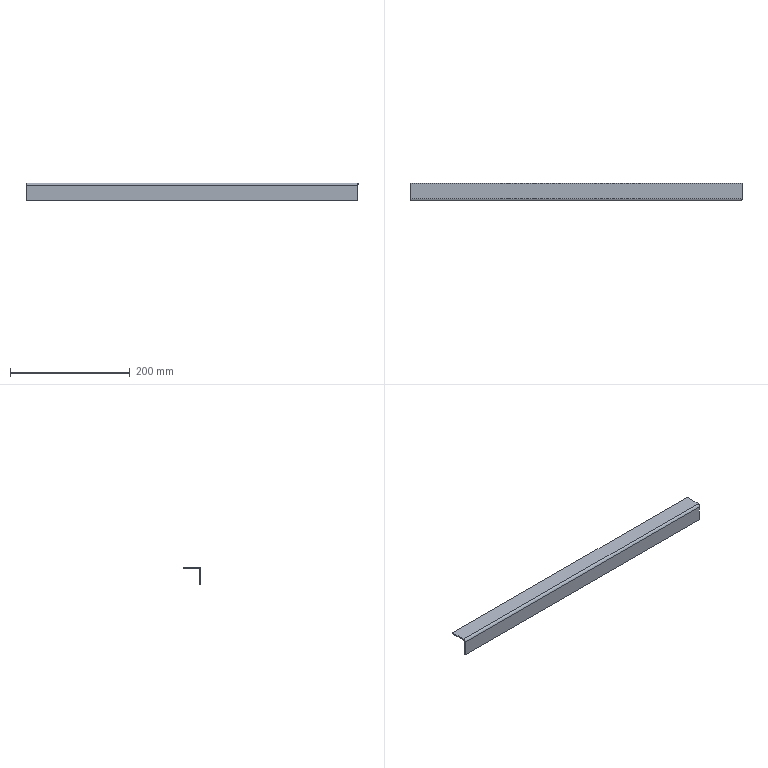Component | SolidWorks | FrontSidePlateAssembly-1_FrontSidePanelReinforcementHorizontalRib-1 | 1 solid | 15 faces | box 555 x 30 x 30 mm | volume 62882 mm3 | plane 13 | cylinder 2 | commonest cylinder face diameters 8 x1 4 x1 | material Plain Carbon Steel
STEP:
#1=CARTESIAN_POINT('',(-8.611,-1.356,52.027));
#2=VERTEX_POINT('',#1);
#3=CARTESIAN_POINT('',(-8.611,-1.278,52.027));
#4=VERTEX_POINT('',#3);
#5=CARTESIAN_POINT('',(-8.611,-1.356,52.027));
#6=DIRECTION('',(0.,1.,0.));
#7=VECTOR('',#6,39.37);
#8=LINE('',#5,#7);
#9=EDGE_CURVE('',#2,#4,#8,.T.);
#10=ORIENTED_EDGE('',*,*,#9,.F.);
#11=CARTESIAN_POINT('',(-8.611,-1.199,52.184));
#12=VERTEX_POINT('',#11);
#13=CARTESIAN_POINT('',(-8.611,-1.199,52.027));
#14=DIRECTION('',(1.,0.,0.));
#15=DIRECTION('',(0.,1.,0.));
#16=AXIS2_PLACEMENT_3D('',#13,#14,#15);
#17=CIRCLE('',#16,0.1575);
#18=EDGE_CURVE('',#12,#2,#17,.T.);
#19=ORIENTED_EDGE('',*,*,#18,.F.);
#20=CARTESIAN_POINT('',(-8.611,-1.199,52.105));
#21=VERTEX_POINT('',#20);
#22=CARTESIAN_POINT('',(-8.611,-1.199,52.105));
#23=DIRECTION('',(0.,0.,1.));
#24=VECTOR('',#23,39.37);
#25=LINE('',#22,#24);
#26=EDGE_CURVE('',#21,#12,#25,.T.);
#27=ORIENTED_EDGE('',*,*,#26,.F.);
#28=CARTESIAN_POINT('',(-8.611,-1.199,52.027));
#29=DIRECTION('',(1.,0.,0.));
#30=DIRECTION('',(0.,1.,0.));
#31=AXIS2_PLACEMENT_3D('',#28,#29,#30);
#32=CIRCLE('',#31,0.07874);
#33=EDGE_CURVE('',#21,#4,#32,.T.);
#34=ORIENTED_EDGE('',*,*,#33,.T.);
#35=EDGE_LOOP('',(#10,#19,#27,#34));
#36=FACE_OUTER_BOUND('',#35,.T.);
#37=CARTESIAN_POINT('',(-8.611,-1.356,52.027));
#38=DIRECTION('',(-1.,0.,0.));
#39=DIRECTION('',(0.,1.,0.));
#40=AXIS2_PLACEMENT_3D('',#37,#38,#39);
#41=PLANE('',#40);
#42=ADVANCED_FACE('',(#36),#41,.T.);
#43=CARTESIAN_POINT('',(-8.611,-1.356,51.003));
#44=VERTEX_POINT('',#43);
#45=CARTESIAN_POINT('',(-8.611,-1.356,52.184));
#46=DIRECTION('',(0.,0.,-1.));
#47=VECTOR('',#46,39.37);
#48=LINE('',#45,#47);
#49=EDGE_CURVE('',#2,#44,#48,.T.);
#50=ORIENTED_EDGE('',*,*,#49,.F.);
#51=ORIENTED_EDGE('',*,*,#9,.T.);
#52=CARTESIAN_POINT('',(-8.611,-1.278,51.003));
#53=VERTEX_POINT('',#52);
#54=CARTESIAN_POINT('',(-8.611,-1.278,52.184));
#55=DIRECTION('',(0.,0.,-1.));
#56=VECTOR('',#55,39.37);
#57=LINE('',#54,#56);
#58=EDGE_CURVE('',#4,#53,#57,.T.);
#59=ORIENTED_EDGE('',*,*,#58,.T.);
#60=CARTESIAN_POINT('',(-8.611,-1.356,51.003));
#61=DIRECTION('',(0.,1.,0.));
#62=VECTOR('',#61,39.37);
#63=LINE('',#60,#62);
#64=EDGE_CURVE('',#44,#53,#63,.T.);
#65=ORIENTED_EDGE('',*,*,#64,.F.);
#66=EDGE_LOOP('',(#50,#51,#59,#65));
#67=FACE_OUTER_BOUND('',#66,.T.);
#68=CARTESIAN_POINT('',(-8.611,-1.199,52.105));
#69=DIRECTION('',(-1.,0.,0.));
#70=DIRECTION('',(0.,1.,0.));
#71=AXIS2_PLACEMENT_3D('',#68,#69,#70);
#72=PLANE('',#71);
#73=ADVANCED_FACE('',(#67),#72,.T.);
#74=CARTESIAN_POINT('',(13.24,-1.27,52.061));
#75=VERTEX_POINT('',#74);
#76=CARTESIAN_POINT('',(13.24,-1.27,52.167));
#77=VERTEX_POINT('',#76);
#78=CARTESIAN_POINT('',(13.24,-1.27,52.184));
#79=DIRECTION('',(0.,0.,1.));
#80=VECTOR('',#79,39.37);
#81=LINE('',#78,#80);
#82=EDGE_CURVE('',#75,#77,#81,.T.);
#83=ORIENTED_EDGE('',*,*,#82,.F.);
#84=CARTESIAN_POINT('',(13.24,-1.199,52.105));
#85=VERTEX_POINT('',#84);
#86=CARTESIAN_POINT('',(13.24,-1.199,52.027));
#87=DIRECTION('',(1.,0.,0.));
#88=DIRECTION('',(0.,1.,0.));
#89=AXIS2_PLACEMENT_3D('',#86,#87,#88);
#90=CIRCLE('',#89,0.07874);
#91=EDGE_CURVE('',#85,#75,#90,.T.);
#92=ORIENTED_EDGE('',*,*,#91,.F.);
#93=CARTESIAN_POINT('',(13.24,-1.199,52.184));
#94=VERTEX_POINT('',#93);
#95=CARTESIAN_POINT('',(13.24,-1.199,52.184));
#96=DIRECTION('',(0.,0.,-1.));
#97=VECTOR('',#96,39.37);
#98=LINE('',#95,#97);
#99=EDGE_CURVE('',#94,#85,#98,.T.);
#100=ORIENTED_EDGE('',*,*,#99,.F.);
#101=CARTESIAN_POINT('',(13.24,-1.199,52.027));
#102=DIRECTION('',(1.,0.,0.));
#103=DIRECTION('',(0.,1.,0.));
#104=AXIS2_PLACEMENT_3D('',#101,#102,#103);
#105=CIRCLE('',#104,0.1575);
#106=EDGE_CURVE('',#94,#77,#105,.T.);
#107=ORIENTED_EDGE('',*,*,#106,.T.);
#108=EDGE_LOOP('',(#83,#92,#100,#107));
#109=FACE_OUTER_BOUND('',#108,.T.);
#110=CARTESIAN_POINT('',(13.24,-1.199,52.184));
#111=DIRECTION('',(1.,0.,0.));
#112=DIRECTION('',(0.,-1.,0.));
#113=AXIS2_PLACEMENT_3D('',#110,#111,#112);
#114=PLANE('',#113);
#115=ADVANCED_FACE('',(#109),#114,.T.);
#116=CARTESIAN_POINT('',(13.24,-0.1752,52.184));
#117=VERTEX_POINT('',#116);
#118=CARTESIAN_POINT('',(13.24,-1.356,52.184));
#119=DIRECTION('',(0.,-1.,0.));
#120=VECTOR('',#119,39.37);
#121=LINE('',#118,#120);
#122=EDGE_CURVE('',#117,#94,#121,.T.);
#123=ORIENTED_EDGE('',*,*,#122,.T.);
#124=ORIENTED_EDGE('',*,*,#99,.T.);
#125=CARTESIAN_POINT('',(13.24,-0.1752,52.105));
#126=VERTEX_POINT('',#125);
#127=CARTESIAN_POINT('',(13.24,-1.356,52.105));
#128=DIRECTION('',(0.,-1.,0.));
#129=VECTOR('',#128,39.37);
#130=LINE('',#127,#129);
#131=EDGE_CURVE('',#126,#85,#130,.T.);
#132=ORIENTED_EDGE('',*,*,#131,.F.);
#133=CARTESIAN_POINT('',(13.24,-0.1752,52.105));
#134=DIRECTION('',(0.,0.,1.));
#135=VECTOR('',#134,39.37);
#136=LINE('',#133,#135);
#137=EDGE_CURVE('',#126,#117,#136,.T.);
#138=ORIENTED_EDGE('',*,*,#137,.T.);
#139=EDGE_LOOP('',(#123,#124,#132,#138));
#140=FACE_OUTER_BOUND('',#139,.T.);
#141=CARTESIAN_POINT('',(13.24,-1.278,52.027));
#142=DIRECTION('',(1.,0.,0.));
#143=DIRECTION('',(0.,-1.,0.));
#144=AXIS2_PLACEMENT_3D('',#141,#142,#143);
#145=PLANE('',#144);
#146=ADVANCED_FACE('',(#140),#145,.T.);
#147=CARTESIAN_POINT('',(13.193,-1.278,52.027));
#148=VERTEX_POINT('',#147);
#149=CARTESIAN_POINT('',(-8.611,-1.278,52.027));
#150=DIRECTION('',(1.,0.,0.));
#151=VECTOR('',#150,39.37);
#152=LINE('',#149,#151);
#153=EDGE_CURVE('',#4,#148,#152,.T.);
#154=ORIENTED_EDGE('',*,*,#153,.T.);
#155=CARTESIAN_POINT('',(13.193,-1.278,51.003));
#156=VERTEX_POINT('',#155);
#157=CARTESIAN_POINT('',(13.193,-1.278,52.184));
#158=DIRECTION('',(0.,0.,-1.));
#159=VECTOR('',#158,39.37);
#160=LINE('',#157,#159);
#161=EDGE_CURVE('',#148,#156,#160,.T.);
#162=ORIENTED_EDGE('',*,*,#161,.T.);
#163=CARTESIAN_POINT('',(-8.611,-1.278,51.003));
#164=DIRECTION('',(1.,0.,0.));
#165=VECTOR('',#164,39.37);
#166=LINE('',#163,#165);
#167=EDGE_CURVE('',#53,#156,#166,.T.);
#168=ORIENTED_EDGE('',*,*,#167,.F.);
#169=ORIENTED_EDGE('',*,*,#58,.F.);
#170=EDGE_LOOP('',(#154,#162,#168,#169));
#171=FACE_OUTER_BOUND('',#170,.T.);
#172=CARTESIAN_POINT('',(-8.611,-1.278,52.184));
#173=DIRECTION('',(0.,-1.,0.));
#174=DIRECTION('',(-1.,0.,0.));
#175=AXIS2_PLACEMENT_3D('',#172,#173,#174);
#176=PLANE('',#175);
#177=ADVANCED_FACE('',(#171),#176,.F.);
#178=CARTESIAN_POINT('',(13.193,-1.356,51.003));
#179=VERTEX_POINT('',#178);
#180=CARTESIAN_POINT('',(13.193,-1.386,51.003));
#181=DIRECTION('',(0.,1.,0.));
#182=VECTOR('',#181,39.37);
#183=LINE('',#180,#182);
#184=EDGE_CURVE('',#179,#156,#183,.T.);
#185=ORIENTED_EDGE('',*,*,#184,.F.);
#186=CARTESIAN_POINT('',(-8.611,-1.356,51.003));
#187=DIRECTION('',(1.,0.,0.));
#188=VECTOR('',#187,39.37);
#189=LINE('',#186,#188);
#190=EDGE_CURVE('',#44,#179,#189,.T.);
#191=ORIENTED_EDGE('',*,*,#190,.F.);
#192=ORIENTED_EDGE('',*,*,#64,.T.);
#193=ORIENTED_EDGE('',*,*,#167,.T.);
#194=EDGE_LOOP('',(#185,#191,#192,#193));
#195=FACE_OUTER_BOUND('',#194,.T.);
#196=CARTESIAN_POINT('',(-8.611,-1.356,51.003));
#197=DIRECTION('',(0.,0.,-1.));
#198=DIRECTION('',(-1.,0.,0.));
#199=AXIS2_PLACEMENT_3D('',#196,#197,#198);
#200=PLANE('',#199);
#201=ADVANCED_FACE('',(#195),#200,.T.);
#202=CARTESIAN_POINT('',(13.193,-1.356,52.027));
#203=VERTEX_POINT('',#202);
#204=CARTESIAN_POINT('',(13.193,-1.356,52.184));
#205=DIRECTION('',(0.,0.,-1.));
#206=VECTOR('',#205,39.37);
#207=LINE('',#204,#206);
#208=EDGE_CURVE('',#203,#179,#207,.T.);
#209=ORIENTED_EDGE('',*,*,#208,.F.);
#210=CARTESIAN_POINT('',(-8.611,-1.356,52.027));
#211=DIRECTION('',(1.,0.,0.));
#212=VECTOR('',#211,39.37);
#213=LINE('',#210,#212);
#214=EDGE_CURVE('',#2,#203,#213,.T.);
#215=ORIENTED_EDGE('',*,*,#214,.F.);
#216=ORIENTED_EDGE('',*,*,#49,.T.);
#217=ORIENTED_EDGE('',*,*,#190,.T.);
#218=EDGE_LOOP('',(#209,#215,#216,#217));
#219=FACE_OUTER_BOUND('',#218,.T.);
#220=CARTESIAN_POINT('',(-8.611,-1.356,52.184));
#221=DIRECTION('',(0.,-1.,0.));
#222=DIRECTION('',(-1.,0.,0.));
#223=AXIS2_PLACEMENT_3D('',#220,#221,#222);
#224=PLANE('',#223);
#225=ADVANCED_FACE('',(#219),#224,.T.);
#226=CARTESIAN_POINT('',(13.193,-1.27,52.167));
#227=VERTEX_POINT('',#226);
#228=CARTESIAN_POINT('',(-8.611,-1.27,52.167));
#229=DIRECTION('',(-1.,0.,0.));
#230=VECTOR('',#229,39.37);
#231=LINE('',#228,#230);
#232=EDGE_CURVE('',#77,#227,#231,.T.);
#233=ORIENTED_EDGE('',*,*,#232,.F.);
#234=ORIENTED_EDGE('',*,*,#106,.F.);
#235=CARTESIAN_POINT('',(-8.611,-1.199,52.184));
#236=DIRECTION('',(1.,0.,0.));
#237=VECTOR('',#236,39.37);
#238=LINE('',#235,#237);
#239=EDGE_CURVE('',#12,#94,#238,.T.);
#240=ORIENTED_EDGE('',*,*,#239,.F.);
#241=ORIENTED_EDGE('',*,*,#18,.T.);
#242=ORIENTED_EDGE('',*,*,#214,.T.);
#243=CARTESIAN_POINT('',(13.193,-1.199,52.027));
#244=DIRECTION('',(1.,0.,0.));
#245=DIRECTION('',(0.,1.,-0.));
#246=AXIS2_PLACEMENT_3D('',#243,#244,#245);
#247=CIRCLE('',#246,0.1575);
#248=EDGE_CURVE('',#227,#203,#247,.T.);
#249=ORIENTED_EDGE('',*,*,#248,.F.);
#250=EDGE_LOOP('',(#233,#234,#240,#241,#242,#249));
#251=FACE_OUTER_BOUND('',#250,.T.);
#252=CARTESIAN_POINT('',(-8.611,-1.199,52.027));
#253=DIRECTION('',(1.,0.,0.));
#254=DIRECTION('',(0.,-1.,0.));
#255=AXIS2_PLACEMENT_3D('',#252,#253,#254);
#256=CYLINDRICAL_SURFACE('',#255,0.1575);
#257=ADVANCED_FACE('',(#251),#256,.T.);
#258=ORIENTED_EDGE('',*,*,#122,.F.);
#259=CARTESIAN_POINT('',(-8.611,-0.1752,52.184));
#260=VERTEX_POINT('',#259);
#261=CARTESIAN_POINT('',(-8.611,-0.1752,52.184));
#262=DIRECTION('',(1.,0.,0.));
#263=VECTOR('',#262,39.37);
#264=LINE('',#261,#263);
#265=EDGE_CURVE('',#260,#117,#264,.T.);
#266=ORIENTED_EDGE('',*,*,#265,.F.);
#267=CARTESIAN_POINT('',(-8.611,-1.356,52.184));
#268=DIRECTION('',(0.,-1.,0.));
#269=VECTOR('',#268,39.37);
#270=LINE('',#267,#269);
#271=EDGE_CURVE('',#260,#12,#270,.T.);
#272=ORIENTED_EDGE('',*,*,#271,.T.);
#273=ORIENTED_EDGE('',*,*,#239,.T.);
#274=EDGE_LOOP('',(#258,#266,#272,#273));
#275=FACE_OUTER_BOUND('',#274,.T.);
#276=CARTESIAN_POINT('',(-8.611,-1.356,52.184));
#277=DIRECTION('',(0.,0.,1.));
#278=DIRECTION('',(1.,0.,0.));
#279=AXIS2_PLACEMENT_3D('',#276,#277,#278);
#280=PLANE('',#279);
#281=ADVANCED_FACE('',(#275),#280,.T.);
#282=ORIENTED_EDGE('',*,*,#137,.F.);
#283=CARTESIAN_POINT('',(-8.611,-0.1752,52.105));
#284=VERTEX_POINT('',#283);
#285=CARTESIAN_POINT('',(-8.611,-0.1752,52.105));
#286=DIRECTION('',(1.,0.,0.));
#287=VECTOR('',#286,39.37);
#288=LINE('',#285,#287);
#289=EDGE_CURVE('',#284,#126,#288,.T.);
#290=ORIENTED_EDGE('',*,*,#289,.F.);
#291=CARTESIAN_POINT('',(-8.611,-0.1752,52.105));
#292=DIRECTION('',(0.,0.,1.));
#293=VECTOR('',#292,39.37);
#294=LINE('',#291,#293);
#295=EDGE_CURVE('',#284,#260,#294,.T.);
#296=ORIENTED_EDGE('',*,*,#295,.T.);
#297=ORIENTED_EDGE('',*,*,#265,.T.);
#298=EDGE_LOOP('',(#282,#290,#296,#297));
#299=FACE_OUTER_BOUND('',#298,.T.);
#300=CARTESIAN_POINT('',(-8.611,-0.1752,52.105));
#301=DIRECTION('',(0.,1.,0.));
#302=DIRECTION('',(1.,0.,0.));
#303=AXIS2_PLACEMENT_3D('',#300,#301,#302);
#304=PLANE('',#303);
#305=ADVANCED_FACE('',(#299),#304,.T.);
#306=ORIENTED_EDGE('',*,*,#131,.T.);
#307=CARTESIAN_POINT('',(-8.611,-1.199,52.105));
#308=DIRECTION('',(1.,0.,0.));
#309=VECTOR('',#308,39.37);
#310=LINE('',#307,#309);
#311=EDGE_CURVE('',#21,#85,#310,.T.);
#312=ORIENTED_EDGE('',*,*,#311,.F.);
#313=CARTESIAN_POINT('',(-8.611,-1.356,52.105));
#314=DIRECTION('',(0.,-1.,0.));
#315=VECTOR('',#314,39.37);
#316=LINE('',#313,#315);
#317=EDGE_CURVE('',#284,#21,#316,.T.);
#318=ORIENTED_EDGE('',*,*,#317,.F.);
#319=ORIENTED_EDGE('',*,*,#289,.T.);
#320=EDGE_LOOP('',(#306,#312,#318,#319));
#321=FACE_OUTER_BOUND('',#320,.T.);
#322=CARTESIAN_POINT('',(-8.611,-1.356,52.105));
#323=DIRECTION('',(0.,0.,1.));
#324=DIRECTION('',(1.,0.,0.));
#325=AXIS2_PLACEMENT_3D('',#322,#323,#324);
#326=PLANE('',#325);
#327=ADVANCED_FACE('',(#321),#326,.F.);
#328=ORIENTED_EDGE('',*,*,#91,.T.);
#329=CARTESIAN_POINT('',(13.193,-1.27,52.061));
#330=VERTEX_POINT('',#329);
#331=CARTESIAN_POINT('',(-8.611,-1.27,52.061));
#332=DIRECTION('',(-1.,0.,0.));
#333=VECTOR('',#332,39.37);
#334=LINE('',#331,#333);
#335=EDGE_CURVE('',#75,#330,#334,.T.);
#336=ORIENTED_EDGE('',*,*,#335,.T.);
#337=CARTESIAN_POINT('',(13.193,-1.199,52.027));
#338=DIRECTION('',(1.,0.,0.));
#339=DIRECTION('',(0.,1.,0.));
#340=AXIS2_PLACEMENT_3D('',#337,#338,#339);
#341=CIRCLE('',#340,0.07874);
#342=EDGE_CURVE('',#330,#148,#341,.T.);
#343=ORIENTED_EDGE('',*,*,#342,.T.);
#344=ORIENTED_EDGE('',*,*,#153,.F.);
#345=ORIENTED_EDGE('',*,*,#33,.F.);
#346=ORIENTED_EDGE('',*,*,#311,.T.);
#347=EDGE_LOOP('',(#328,#336,#343,#344,#345,#346));
#348=FACE_OUTER_BOUND('',#347,.T.);
#349=CARTESIAN_POINT('',(-8.611,-1.199,52.027));
#350=DIRECTION('',(1.,0.,0.));
#351=DIRECTION('',(0.,-1.,0.));
#352=AXIS2_PLACEMENT_3D('',#349,#350,#351);
#353=CYLINDRICAL_SURFACE('',#352,0.07874);
#354=ADVANCED_FACE('',(#348),#353,.F.);
#355=ORIENTED_EDGE('',*,*,#317,.T.);
#356=ORIENTED_EDGE('',*,*,#26,.T.);
#357=ORIENTED_EDGE('',*,*,#271,.F.);
#358=ORIENTED_EDGE('',*,*,#295,.F.);
#359=EDGE_LOOP('',(#355,#356,#357,#358));
#360=FACE_OUTER_BOUND('',#359,.T.);
#361=CARTESIAN_POINT('',(-8.611,-1.199,52.027));
#362=DIRECTION('',(-1.,0.,0.));
#363=DIRECTION('',(0.,1.,0.));
#364=AXIS2_PLACEMENT_3D('',#361,#362,#363);
#365=PLANE('',#364);
#366=ADVANCED_FACE('',(#360),#365,.T.);
#367=ORIENTED_EDGE('',*,*,#208,.T.);
#368=ORIENTED_EDGE('',*,*,#184,.T.);
#369=ORIENTED_EDGE('',*,*,#161,.F.);
#370=ORIENTED_EDGE('',*,*,#342,.F.);
#371=CARTESIAN_POINT('',(13.193,-1.27,52.184));
#372=DIRECTION('',(0.,0.,-1.));
#373=VECTOR('',#372,39.37);
#374=LINE('',#371,#373);
#375=EDGE_CURVE('',#227,#330,#374,.T.);
#376=ORIENTED_EDGE('',*,*,#375,.F.);
#377=ORIENTED_EDGE('',*,*,#248,.T.);
#378=EDGE_LOOP('',(#367,#368,#369,#370,#376,#377));
#379=FACE_OUTER_BOUND('',#378,.T.);
#380=CARTESIAN_POINT('',(13.193,-1.386,52.184));
#381=DIRECTION('',(-1.,0.,0.));
#382=DIRECTION('',(0.,1.,0.));
#383=AXIS2_PLACEMENT_3D('',#380,#381,#382);
#384=PLANE('',#383);
#385=ADVANCED_FACE('',(#379),#384,.F.);
#386=ORIENTED_EDGE('',*,*,#232,.T.);
#387=ORIENTED_EDGE('',*,*,#375,.T.);
#388=ORIENTED_EDGE('',*,*,#335,.F.);
#389=ORIENTED_EDGE('',*,*,#82,.T.);
#390=EDGE_LOOP('',(#386,#387,#388,#389));
#391=FACE_OUTER_BOUND('',#390,.T.);
#392=CARTESIAN_POINT('',(13.276,-1.27,52.184));
#393=DIRECTION('',(0.,1.,0.));
#394=DIRECTION('',(1.,0.,0.));
#395=AXIS2_PLACEMENT_3D('',#392,#393,#394);
#396=PLANE('',#395);
#397=ADVANCED_FACE('',(#391),#396,.F.);
#398=CLOSED_SHELL('',(#42,#73,#115,#146,#177,#201,#225,#257,#281,#305,#327,#354,#366,#385,#397));
#399=MANIFOLD_SOLID_BREP('',#398);
#400=CARTESIAN_POINT('',(0.,0.,0.));
#401=DIRECTION('',(0.,0.,1.));
#402=DIRECTION('',(1.,0.,0.));
#403=AXIS2_PLACEMENT_3D('',#400,#401,#402);
#404=(LENGTH_UNIT()NAMED_UNIT(*)SI_UNIT($,.METRE.));
#405=LENGTH_MEASURE_WITH_UNIT(LENGTH_MEASURE(0.0254),#404);
#406=DIMENSIONAL_EXPONENTS(1.,0.,0.,0.,0.,0.,0.);
#407=(CONVERSION_BASED_UNIT('',#405)LENGTH_UNIT()NAMED_UNIT(#406));
#408=UNCERTAINTY_MEASURE_WITH_UNIT(LENGTH_MEASURE(0.00001),#407,'','');
#409=(NAMED_UNIT(*)PLANE_ANGLE_UNIT()SI_UNIT($,.RADIAN.));
#410=(NAMED_UNIT(*)SI_UNIT($,.STERADIAN.)SOLID_ANGLE_UNIT());
#411=(GEOMETRIC_REPRESENTATION_CONTEXT(3)GLOBAL_UNCERTAINTY_ASSIGNED_CONTEXT((#408))GLOBAL_UNIT_ASSIGNED_CONTEXT((#407,#409,#410))REPRESENTATION_CONTEXT('',''));
#412=ADVANCED_BREP_SHAPE_REPRESENTATION('',(#399,#403),#411);
#413=COLOUR_RGB('',0.7922,0.8196,0.9333);
#414=FILL_AREA_STYLE_COLOUR('',#413);
#415=FILL_AREA_STYLE('',(#414));
#416=SURFACE_STYLE_FILL_AREA(#415);
#417=SURFACE_SIDE_STYLE('',(#416));
#418=SURFACE_STYLE_USAGE(.BOTH.,#417);
#419=PRESENTATION_STYLE_ASSIGNMENT((#418));
#420=STYLED_ITEM('',(#419),#399);
#421=PRESENTATION_LAYER_ASSIGNMENT('','',(#420));
#422=(LENGTH_UNIT()NAMED_UNIT(*)SI_UNIT($,.METRE.));
#423=LENGTH_MEASURE_WITH_UNIT(LENGTH_MEASURE(0.0254),#422);
#424=DIMENSIONAL_EXPONENTS(1.,0.,0.,0.,0.,0.,0.);
#425=(CONVERSION_BASED_UNIT('',#423)LENGTH_UNIT()NAMED_UNIT(#424));
#426=UNCERTAINTY_MEASURE_WITH_UNIT(LENGTH_MEASURE(0.00001),#425,'','');
#427=(NAMED_UNIT(*)PLANE_ANGLE_UNIT()SI_UNIT($,.RADIAN.));
#428=(NAMED_UNIT(*)SI_UNIT($,.STERADIAN.)SOLID_ANGLE_UNIT());
#429=(GEOMETRIC_REPRESENTATION_CONTEXT(3)GLOBAL_UNCERTAINTY_ASSIGNED_CONTEXT((#426))GLOBAL_UNIT_ASSIGNED_CONTEXT((#425,#427,#428))REPRESENTATION_CONTEXT('',''));
#430=MECHANICAL_DESIGN_GEOMETRIC_PRESENTATION_REPRESENTATION('',(#420),#429);